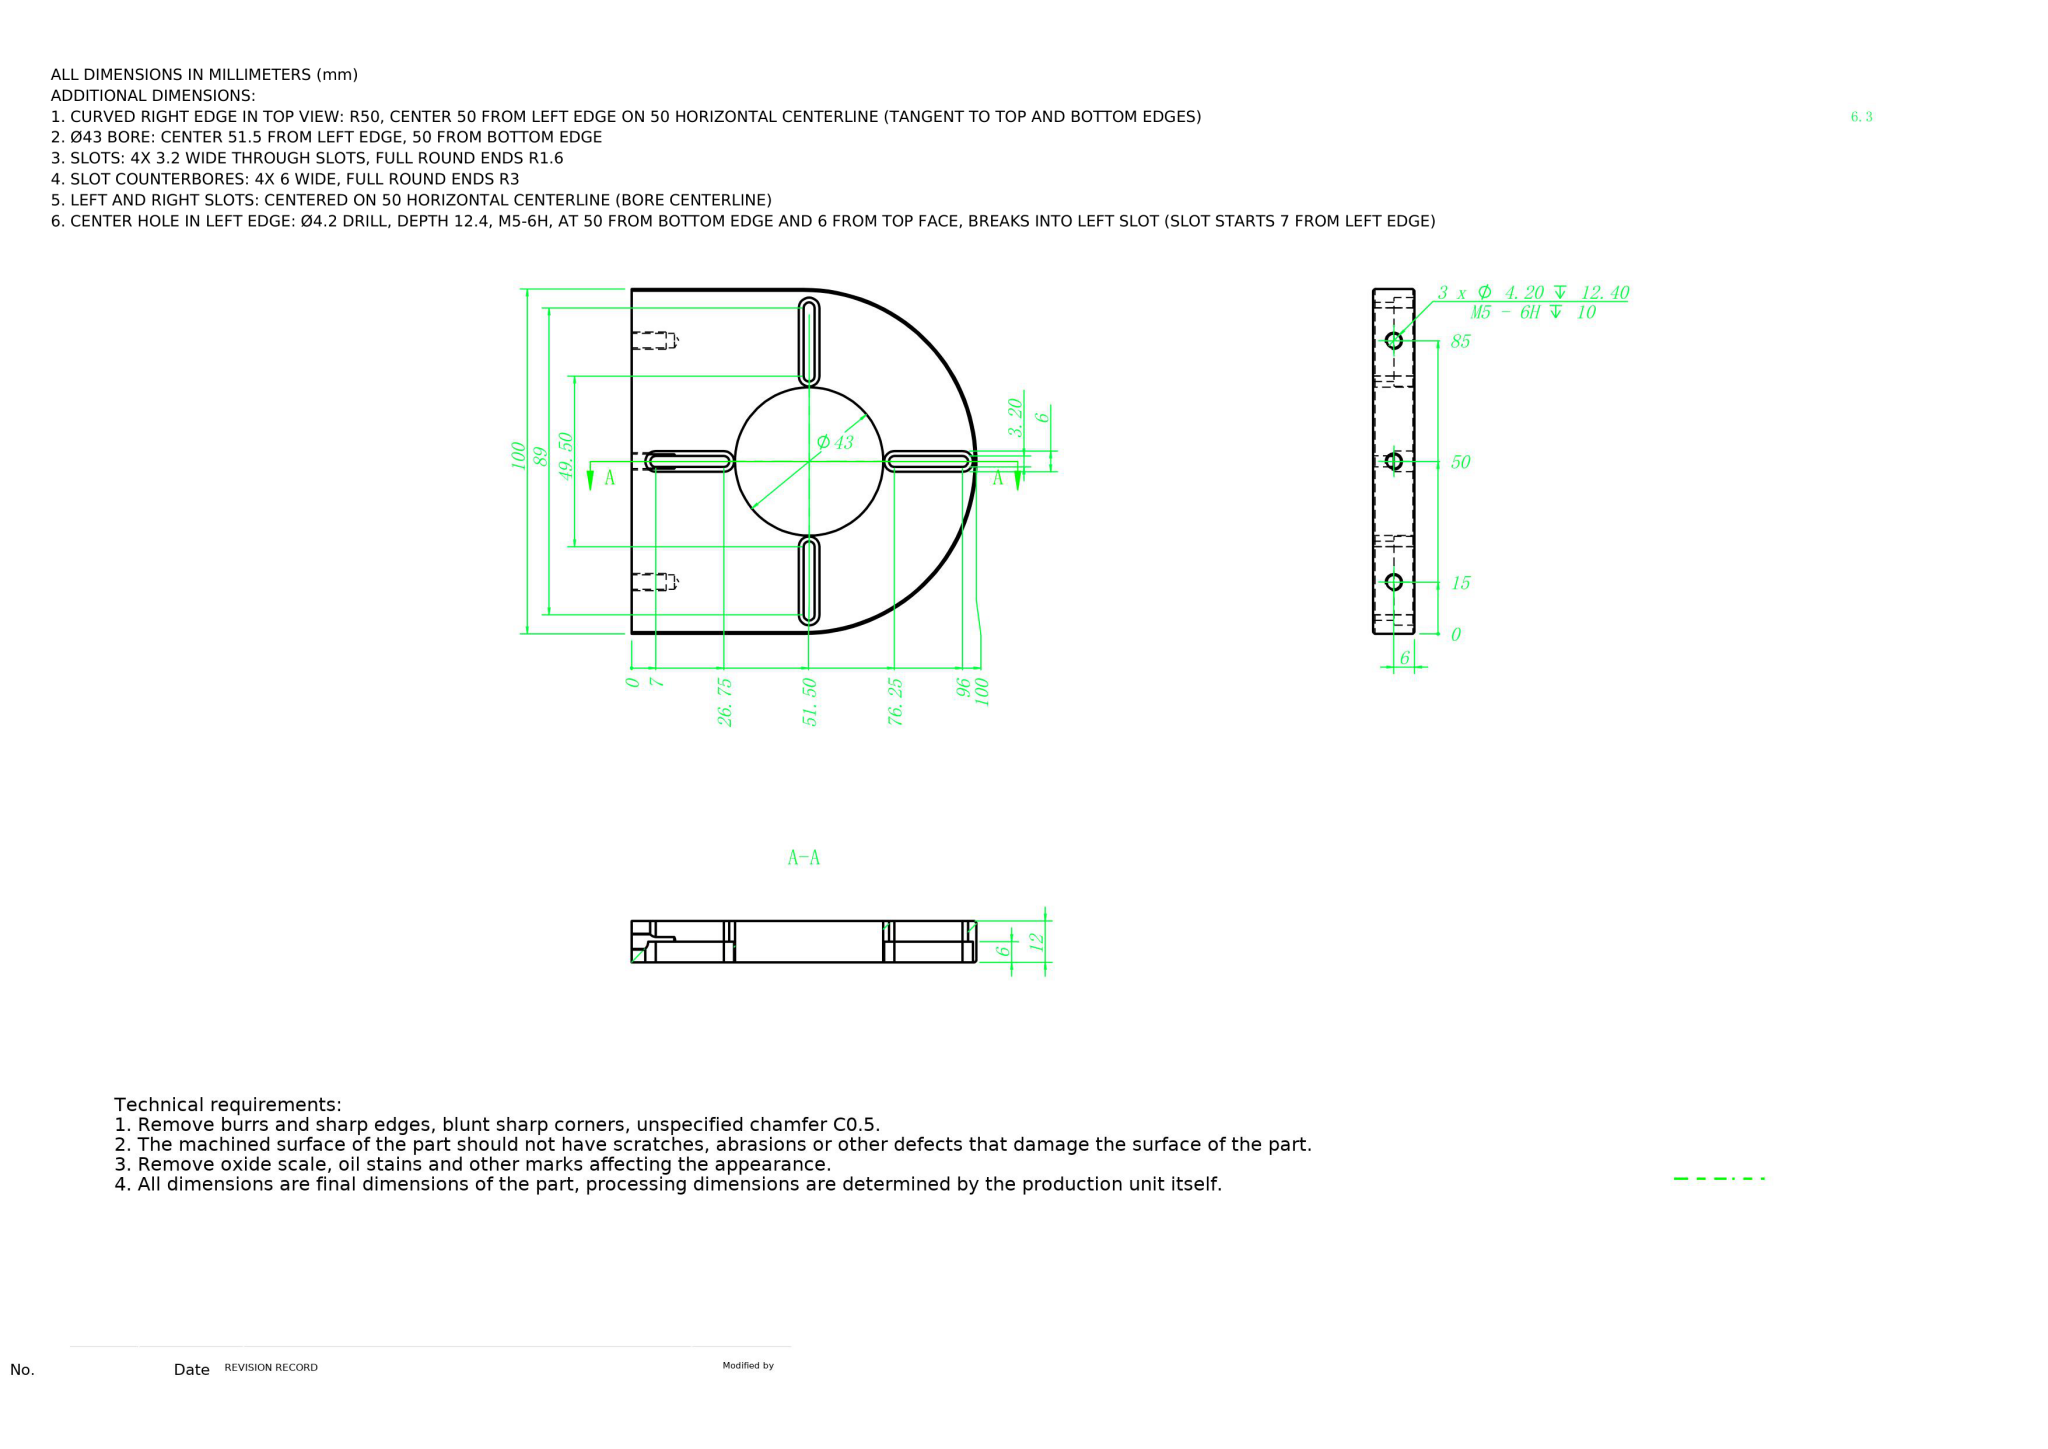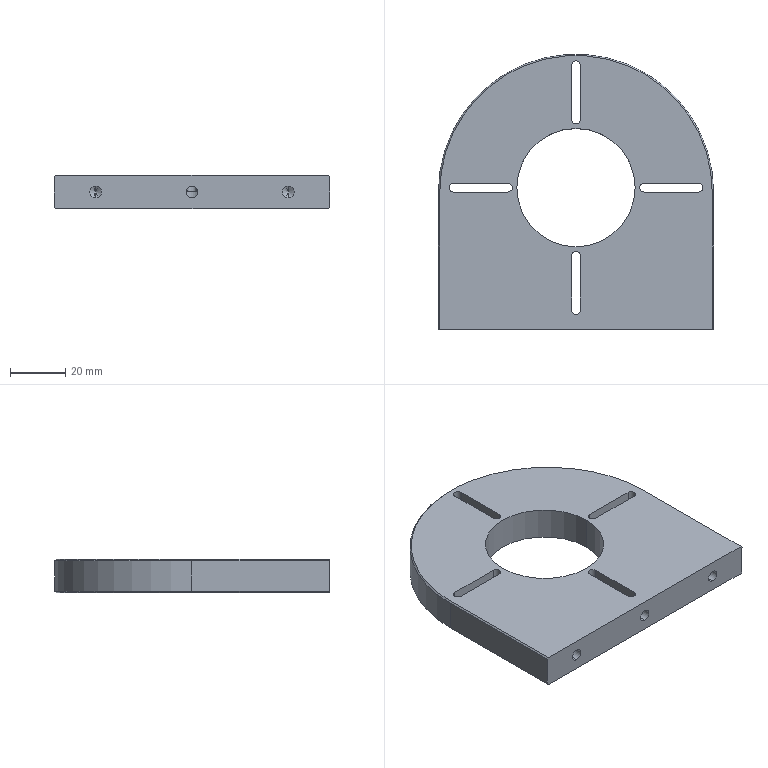Part | NX | mm | 1 solid | 66 faces | box 100 x 100 x 12 mm | volume 83971 mm3 | cylinder 29 | plane 29 | cone 8 | commonest cylinder face diameters 3.2 x10 6 x10 4.2 x6 43 x2 100 x1